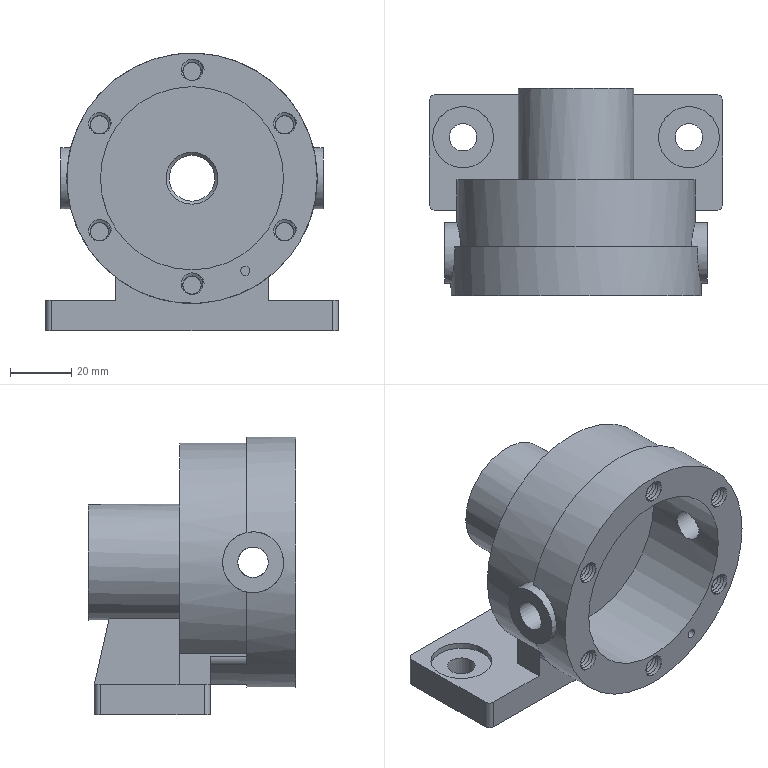Component | NX | PUMP_BODY | 1 solid | 112 faces | volume 169420 mm3 | plane 45 | cylinder 39 | spline 27 | cone 1 | commonest cylinder face diameters 6 x8 4 x7 8 x6 20 x4 5 x3 10 x2 9 x2 60 x1